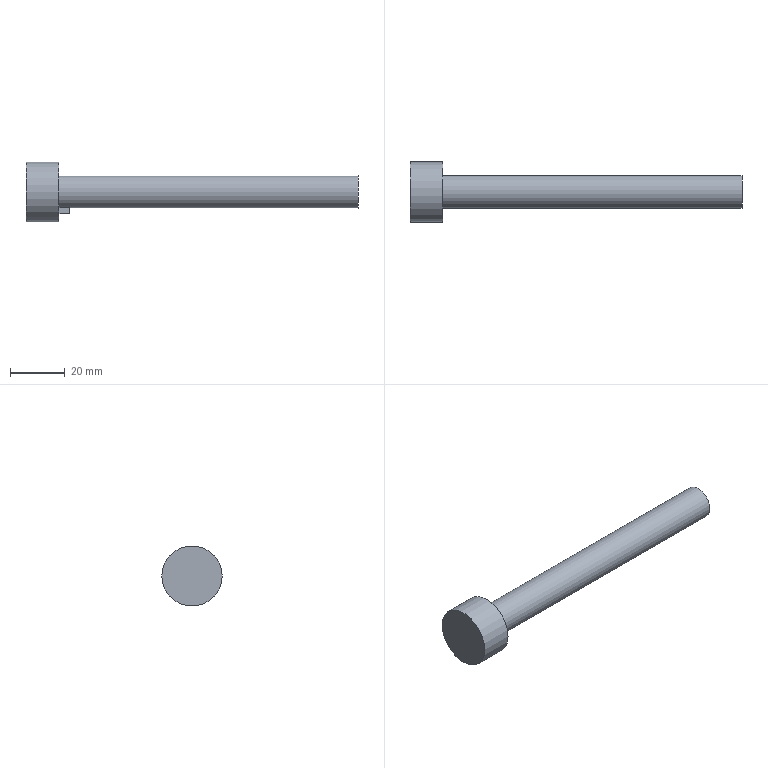Component | NX | BOLT_M12 | 2 solids | 11 faces | box 121 x 22 x 22 mm | volume 16923 mm3 | plane 8 | cylinder 3 | commonest cylinder face diameters 12 x2 22 x1
STEP:
#1=CARTESIAN_POINT('',(0.,0.,0.));
#2=DIRECTION('',(0.,0.,1.));
#3=DIRECTION('',(1.,0.,0.));
#4=AXIS2_PLACEMENT_3D('',#1,#2,#3);
#5=CARTESIAN_POINT('',(16.,11.,-95.));
#6=VERTEX_POINT('',#5);
#7=CARTESIAN_POINT('',(16.,0.,-95.));
#8=DIRECTION('',(-1.,0.,0.));
#9=DIRECTION('',(0.,1.,0.));
#10=AXIS2_PLACEMENT_3D('',#7,#8,#9);
#11=CIRCLE('',#10,11.);
#12=CARTESIAN_POINT('',(16.,0.,-95.));
#13=DIRECTION('',(-1.,0.,0.));
#14=DIRECTION('',(0.,0.,1.));
#15=AXIS2_PLACEMENT_3D('',#12,#13,#14);
#16=PLANE('',#15);
#17=CARTESIAN_POINT('',(0.,0.));
#18=DIRECTION('',(0.,1.));
#19=AXIS2_PLACEMENT_2D('',#17,#18);
#20=CIRCLE('',#19,11.);
#21=(GEOMETRIC_REPRESENTATION_CONTEXT(2)PARAMETRIC_REPRESENTATION_CONTEXT()REPRESENTATION_CONTEXT('',''));
#22=DEFINITIONAL_REPRESENTATION('',(#20),#21);
#23=PCURVE('',#16,#22);
#24=CARTESIAN_POINT('',(4.,0.,-95.));
#25=DIRECTION('',(1.,0.,0.));
#26=DIRECTION('',(0.,0.,-1.));
#27=AXIS2_PLACEMENT_3D('',#24,#25,#26);
#28=CYLINDRICAL_SURFACE('',#27,11.);
#29=CARTESIAN_POINT('',(7.854,12.));
#30=DIRECTION('',(-1.,0.));
#31=VECTOR('',#30,1.);
#32=LINE('',#29,#31);
#33=(GEOMETRIC_REPRESENTATION_CONTEXT(2)PARAMETRIC_REPRESENTATION_CONTEXT()REPRESENTATION_CONTEXT('',''));
#34=DEFINITIONAL_REPRESENTATION('',(#32),#33);
#35=PCURVE('',#28,#34);
#36=SURFACE_CURVE('',#11,(#23,#35),.PCURVE_S1.);
#37=EDGE_CURVE('',#6,#6,#36,.T.);
#38=ORIENTED_EDGE('',*,*,#37,.F.);
#39=EDGE_LOOP('',(#38));
#40=FACE_BOUND('',#39,.T.);
#41=CARTESIAN_POINT('',(16.,6.,-95.));
#42=VERTEX_POINT('',#41);
#43=CARTESIAN_POINT('',(16.,0.,-95.));
#44=DIRECTION('',(1.,0.,0.));
#45=DIRECTION('',(0.,1.,0.));
#46=AXIS2_PLACEMENT_3D('',#43,#44,#45);
#47=CIRCLE('',#46,6.);
#48=CARTESIAN_POINT('',(0.,6.));
#49=CARTESIAN_POINT('',(10.392,6.));
#50=CARTESIAN_POINT('',(5.196,-3.));
#51=CARTESIAN_POINT('',(0.,-12.));
#52=CARTESIAN_POINT('',(-5.196,-3.));
#53=CARTESIAN_POINT('',(-10.392,6.));
#54=CARTESIAN_POINT('',(0.,6.));
#55=(BOUNDED_CURVE()B_SPLINE_CURVE(2,(#48,#49,#50,#51,#52,#53,#54),.UNSPECIFIED.,.T.,.F.)B_SPLINE_CURVE_WITH_KNOTS((1,2,2,2,2,1),(-2.094,0.,2.094,4.189,6.283,8.378),.UNSPECIFIED.)CURVE()GEOMETRIC_REPRESENTATION_ITEM()RATIONAL_B_SPLINE_CURVE((1.,0.5,1.,0.5,1.,0.5,1.))REPRESENTATION_ITEM(''));
#56=(GEOMETRIC_REPRESENTATION_CONTEXT(2)PARAMETRIC_REPRESENTATION_CONTEXT()REPRESENTATION_CONTEXT('',''));
#57=DEFINITIONAL_REPRESENTATION('',(#55),#56);
#58=PCURVE('',#16,#57);
#59=CARTESIAN_POINT('',(125.,0.,-95.));
#60=DIRECTION('',(-1.,0.,0.));
#61=DIRECTION('',(0.,0.,1.));
#62=AXIS2_PLACEMENT_3D('',#59,#60,#61);
#63=CYLINDRICAL_SURFACE('',#62,6.);
#64=CARTESIAN_POINT('',(7.854,109.));
#65=DIRECTION('',(-1.,0.));
#66=VECTOR('',#65,1.);
#67=LINE('',#64,#66);
#68=(GEOMETRIC_REPRESENTATION_CONTEXT(2)PARAMETRIC_REPRESENTATION_CONTEXT()REPRESENTATION_CONTEXT('',''));
#69=DEFINITIONAL_REPRESENTATION('',(#67),#68);
#70=PCURVE('',#63,#69);
#71=SURFACE_CURVE('',#47,(#58,#70),.PCURVE_S1.);
#72=EDGE_CURVE('',#42,#42,#71,.T.);
#73=ORIENTED_EDGE('',*,*,#72,.F.);
#74=EDGE_LOOP('',(#73));
#75=FACE_BOUND('',#74,.T.);
#76=ADVANCED_FACE('',(#40,#75),#16,.F.);
#77=CARTESIAN_POINT('',(4.,11.,-95.));
#78=VERTEX_POINT('',#77);
#79=CARTESIAN_POINT('',(4.,0.,-95.));
#80=DIRECTION('',(-1.,0.,0.));
#81=DIRECTION('',(0.,1.,0.));
#82=AXIS2_PLACEMENT_3D('',#79,#80,#81);
#83=CIRCLE('',#82,11.);
#84=CARTESIAN_POINT('',(7.854,0.));
#85=DIRECTION('',(-1.,0.));
#86=VECTOR('',#85,1.);
#87=LINE('',#84,#86);
#88=(GEOMETRIC_REPRESENTATION_CONTEXT(2)PARAMETRIC_REPRESENTATION_CONTEXT()REPRESENTATION_CONTEXT('',''));
#89=DEFINITIONAL_REPRESENTATION('',(#87),#88);
#90=PCURVE('',#28,#89);
#91=CARTESIAN_POINT('',(4.,0.,-95.));
#92=DIRECTION('',(-1.,0.,0.));
#93=DIRECTION('',(0.,0.,1.));
#94=AXIS2_PLACEMENT_3D('',#91,#92,#93);
#95=PLANE('',#94);
#96=CARTESIAN_POINT('',(0.,0.));
#97=DIRECTION('',(0.,1.));
#98=AXIS2_PLACEMENT_2D('',#96,#97);
#99=CIRCLE('',#98,11.);
#100=(GEOMETRIC_REPRESENTATION_CONTEXT(2)PARAMETRIC_REPRESENTATION_CONTEXT()REPRESENTATION_CONTEXT('',''));
#101=DEFINITIONAL_REPRESENTATION('',(#99),#100);
#102=PCURVE('',#95,#101);
#103=SURFACE_CURVE('',#83,(#90,#102),.PCURVE_S1.);
#104=EDGE_CURVE('',#78,#78,#103,.T.);
#105=ORIENTED_EDGE('',*,*,#104,.F.);
#106=CARTESIAN_POINT('',(4.,11.,-95.));
#107=CARTESIAN_POINT('',(16.,11.,-95.));
#108=B_SPLINE_CURVE_WITH_KNOTS('',1,(#106,#107),.UNSPECIFIED.,.F.,.F.,(2,2),(0.,12.),.PIECEWISE_BEZIER_KNOTS.);
#109=CARTESIAN_POINT('',(7.854,0.));
#110=DIRECTION('',(0.,1.));
#111=VECTOR('',#110,1.);
#112=LINE('',#109,#111);
#113=(GEOMETRIC_REPRESENTATION_CONTEXT(2)PARAMETRIC_REPRESENTATION_CONTEXT()REPRESENTATION_CONTEXT('',''));
#114=DEFINITIONAL_REPRESENTATION('',(#112),#113);
#115=PCURVE('',#28,#114);
#116=CARTESIAN_POINT('',(1.571,0.));
#117=DIRECTION('',(0.,1.));
#118=VECTOR('',#117,1.);
#119=LINE('',#116,#118);
#120=(GEOMETRIC_REPRESENTATION_CONTEXT(2)PARAMETRIC_REPRESENTATION_CONTEXT()REPRESENTATION_CONTEXT('',''));
#121=DEFINITIONAL_REPRESENTATION('',(#119),#120);
#122=PCURVE('',#28,#121);
#123=SEAM_CURVE('',#108,(#115,#122),.PCURVE_S1.);
#124=EDGE_CURVE('',#78,#6,#123,.T.);
#125=ORIENTED_EDGE('',*,*,#124,.T.);
#126=ORIENTED_EDGE('',*,*,#37,.T.);
#127=ORIENTED_EDGE('',*,*,#124,.F.);
#128=EDGE_LOOP('',(#105,#125,#126,#127));
#129=FACE_BOUND('',#128,.T.);
#130=ADVANCED_FACE('',(#129),#28,.T.);
#131=ORIENTED_EDGE('',*,*,#104,.T.);
#132=EDGE_LOOP('',(#131));
#133=FACE_BOUND('',#132,.T.);
#134=ADVANCED_FACE('',(#133),#95,.T.);
#135=CARTESIAN_POINT('',(125.,6.,-95.));
#136=VERTEX_POINT('',#135);
#137=CARTESIAN_POINT('',(125.,0.,-95.));
#138=DIRECTION('',(1.,0.,0.));
#139=DIRECTION('',(0.,1.,0.));
#140=AXIS2_PLACEMENT_3D('',#137,#138,#139);
#141=CIRCLE('',#140,6.);
#142=CARTESIAN_POINT('',(7.854,0.));
#143=DIRECTION('',(-1.,0.));
#144=VECTOR('',#143,1.);
#145=LINE('',#142,#144);
#146=(GEOMETRIC_REPRESENTATION_CONTEXT(2)PARAMETRIC_REPRESENTATION_CONTEXT()REPRESENTATION_CONTEXT('',''));
#147=DEFINITIONAL_REPRESENTATION('',(#145),#146);
#148=PCURVE('',#63,#147);
#149=CARTESIAN_POINT('',(125.,0.,-95.));
#150=DIRECTION('',(1.,0.,0.));
#151=DIRECTION('',(0.,0.,-1.));
#152=AXIS2_PLACEMENT_3D('',#149,#150,#151);
#153=PLANE('',#152);
#154=CARTESIAN_POINT('',(0.,0.));
#155=DIRECTION('',(0.,1.));
#156=AXIS2_PLACEMENT_2D('',#154,#155);
#157=CIRCLE('',#156,6.);
#158=(GEOMETRIC_REPRESENTATION_CONTEXT(2)PARAMETRIC_REPRESENTATION_CONTEXT()REPRESENTATION_CONTEXT('',''));
#159=DEFINITIONAL_REPRESENTATION('',(#157),#158);
#160=PCURVE('',#153,#159);
#161=SURFACE_CURVE('',#141,(#148,#160),.PCURVE_S1.);
#162=EDGE_CURVE('',#136,#136,#161,.T.);
#163=ORIENTED_EDGE('',*,*,#162,.F.);
#164=CARTESIAN_POINT('',(125.,6.,-95.));
#165=CARTESIAN_POINT('',(16.,6.,-95.));
#166=B_SPLINE_CURVE_WITH_KNOTS('',1,(#164,#165),.UNSPECIFIED.,.F.,.F.,(2,2),(0.,109.),.PIECEWISE_BEZIER_KNOTS.);
#167=CARTESIAN_POINT('',(7.854,0.));
#168=DIRECTION('',(0.,1.));
#169=VECTOR('',#168,1.);
#170=LINE('',#167,#169);
#171=(GEOMETRIC_REPRESENTATION_CONTEXT(2)PARAMETRIC_REPRESENTATION_CONTEXT()REPRESENTATION_CONTEXT('',''));
#172=DEFINITIONAL_REPRESENTATION('',(#170),#171);
#173=PCURVE('',#63,#172);
#174=CARTESIAN_POINT('',(1.571,0.));
#175=DIRECTION('',(0.,1.));
#176=VECTOR('',#175,1.);
#177=LINE('',#174,#176);
#178=(GEOMETRIC_REPRESENTATION_CONTEXT(2)PARAMETRIC_REPRESENTATION_CONTEXT()REPRESENTATION_CONTEXT('',''));
#179=DEFINITIONAL_REPRESENTATION('',(#177),#178);
#180=PCURVE('',#63,#179);
#181=SEAM_CURVE('',#166,(#173,#180),.PCURVE_S1.);
#182=EDGE_CURVE('',#136,#42,#181,.T.);
#183=ORIENTED_EDGE('',*,*,#182,.T.);
#184=ORIENTED_EDGE('',*,*,#72,.T.);
#185=ORIENTED_EDGE('',*,*,#182,.F.);
#186=EDGE_LOOP('',(#163,#183,#184,#185));
#187=FACE_BOUND('',#186,.T.);
#188=ADVANCED_FACE('',(#187),#63,.T.);
#189=ORIENTED_EDGE('',*,*,#162,.T.);
#190=EDGE_LOOP('',(#189));
#191=FACE_BOUND('',#190,.T.);
#192=ADVANCED_FACE('',(#191),#153,.T.);
#193=CLOSED_SHELL('',(#76,#130,#134,#188,#192));
#194=MANIFOLD_SOLID_BREP('',#193);
#195=(LENGTH_UNIT()NAMED_UNIT(*)SI_UNIT(.MILLI.,.METRE.));
#196=UNCERTAINTY_MEASURE_WITH_UNIT(LENGTH_MEASURE(0.00001),#195,'','');
#197=(NAMED_UNIT(*)PLANE_ANGLE_UNIT()SI_UNIT($,.RADIAN.));
#198=(NAMED_UNIT(*)SI_UNIT($,.STERADIAN.)SOLID_ANGLE_UNIT());
#199=(GEOMETRIC_REPRESENTATION_CONTEXT(3)GLOBAL_UNCERTAINTY_ASSIGNED_CONTEXT((#196))GLOBAL_UNIT_ASSIGNED_CONTEXT((#195,#197,#198))REPRESENTATION_CONTEXT('',''));
#200=ADVANCED_BREP_SHAPE_REPRESENTATION('',(#4,#194),#199);
#201=CARTESIAN_POINT('',(0.,0.,0.));
#202=DIRECTION('',(0.,0.,1.));
#203=DIRECTION('',(1.,0.,0.));
#204=AXIS2_PLACEMENT_3D('',#201,#202,#203);
#205=CARTESIAN_POINT('',(0.,0.,0.));
#206=DIRECTION('',(0.,0.,1.));
#207=DIRECTION('',(1.,0.,0.));
#208=AXIS2_PLACEMENT_3D('',#205,#206,#207);
#209=(LENGTH_UNIT()NAMED_UNIT(*)SI_UNIT(.MILLI.,.METRE.));
#210=UNCERTAINTY_MEASURE_WITH_UNIT(LENGTH_MEASURE(0.000002),#209,'','');
#211=(NAMED_UNIT(*)PLANE_ANGLE_UNIT()SI_UNIT($,.RADIAN.));
#212=(NAMED_UNIT(*)SI_UNIT($,.STERADIAN.)SOLID_ANGLE_UNIT());
#213=(GEOMETRIC_REPRESENTATION_CONTEXT(3)GLOBAL_UNCERTAINTY_ASSIGNED_CONTEXT((#210))GLOBAL_UNIT_ASSIGNED_CONTEXT((#209,#211,#212))REPRESENTATION_CONTEXT('',''));
#214=SHAPE_REPRESENTATION('',(#4,#204,#208),#213);
#215=ITEM_DEFINED_TRANSFORMATION('','',#4,#204);
#216=(REPRESENTATION_RELATIONSHIP('','',#200,#214)REPRESENTATION_RELATIONSHIP_WITH_TRANSFORMATION(#215)SHAPE_REPRESENTATION_RELATIONSHIP());
#217=CARTESIAN_POINT('',(16.,-2.,-103.));
#218=VERTEX_POINT('',#217);
#219=CARTESIAN_POINT('',(16.,-2.,-100.657));
#220=VERTEX_POINT('',#219);
#221=CARTESIAN_POINT('',(16.,-2.,-103.));
#222=DIRECTION('',(0.,0.,1.));
#223=VECTOR('',#222,1.);
#224=LINE('',#221,#223);
#225=CARTESIAN_POINT('',(20.,-2.,-103.));
#226=DIRECTION('',(0.,-1.,0.));
#227=DIRECTION('',(0.,0.,1.));
#228=AXIS2_PLACEMENT_3D('',#225,#226,#227);
#229=PLANE('',#228);
#230=CARTESIAN_POINT('',(0.,4.));
#231=DIRECTION('',(1.,0.));
#232=VECTOR('',#231,1.);
#233=LINE('',#230,#232);
#234=(GEOMETRIC_REPRESENTATION_CONTEXT(2)PARAMETRIC_REPRESENTATION_CONTEXT()REPRESENTATION_CONTEXT('',''));
#235=DEFINITIONAL_REPRESENTATION('',(#233),#234);
#236=PCURVE('',#229,#235);
#237=CARTESIAN_POINT('',(16.,0.,-95.));
#238=DIRECTION('',(1.,0.,0.));
#239=DIRECTION('',(0.,0.,-1.));
#240=AXIS2_PLACEMENT_3D('',#237,#238,#239);
#241=PLANE('',#240);
#242=CARTESIAN_POINT('',(8.,-2.));
#243=DIRECTION('',(-1.,0.));
#244=VECTOR('',#243,1.);
#245=LINE('',#242,#244);
#246=(GEOMETRIC_REPRESENTATION_CONTEXT(2)PARAMETRIC_REPRESENTATION_CONTEXT()REPRESENTATION_CONTEXT('',''));
#247=DEFINITIONAL_REPRESENTATION('',(#245),#246);
#248=PCURVE('',#241,#247);
#249=SURFACE_CURVE('',#224,(#236,#248),.PCURVE_S1.);
#250=EDGE_CURVE('',#218,#220,#249,.T.);
#251=ORIENTED_EDGE('',*,*,#250,.F.);
#252=CARTESIAN_POINT('',(20.,-2.,-103.));
#253=VERTEX_POINT('',#252);
#254=CARTESIAN_POINT('',(20.,-2.,-103.));
#255=DIRECTION('',(-1.,0.,0.));
#256=VECTOR('',#255,1.);
#257=LINE('',#254,#256);
#258=CARTESIAN_POINT('',(0.,0.));
#259=DIRECTION('',(0.,1.));
#260=VECTOR('',#259,1.);
#261=LINE('',#258,#260);
#262=(GEOMETRIC_REPRESENTATION_CONTEXT(2)PARAMETRIC_REPRESENTATION_CONTEXT()REPRESENTATION_CONTEXT('',''));
#263=DEFINITIONAL_REPRESENTATION('',(#261),#262);
#264=PCURVE('',#229,#263);
#265=CARTESIAN_POINT('',(20.,2.,-103.));
#266=DIRECTION('',(0.,0.,-1.));
#267=DIRECTION('',(-1.,0.,0.));
#268=AXIS2_PLACEMENT_3D('',#265,#266,#267);
#269=PLANE('',#268);
#270=CARTESIAN_POINT('',(0.,-4.));
#271=DIRECTION('',(1.,0.));
#272=VECTOR('',#271,1.);
#273=LINE('',#270,#272);
#274=(GEOMETRIC_REPRESENTATION_CONTEXT(2)PARAMETRIC_REPRESENTATION_CONTEXT()REPRESENTATION_CONTEXT('',''));
#275=DEFINITIONAL_REPRESENTATION('',(#273),#274);
#276=PCURVE('',#269,#275);
#277=SURFACE_CURVE('',#257,(#264,#276),.PCURVE_S1.);
#278=EDGE_CURVE('',#253,#218,#277,.T.);
#279=ORIENTED_EDGE('',*,*,#278,.F.);
#280=CARTESIAN_POINT('',(20.,-2.,-100.657));
#281=VERTEX_POINT('',#280);
#282=CARTESIAN_POINT('',(20.,-2.,-103.));
#283=DIRECTION('',(0.,0.,1.));
#284=VECTOR('',#283,1.);
#285=LINE('',#282,#284);
#286=CARTESIAN_POINT('',(0.,0.));
#287=DIRECTION('',(1.,0.));
#288=VECTOR('',#287,1.);
#289=LINE('',#286,#288);
#290=(GEOMETRIC_REPRESENTATION_CONTEXT(2)PARAMETRIC_REPRESENTATION_CONTEXT()REPRESENTATION_CONTEXT('',''));
#291=DEFINITIONAL_REPRESENTATION('',(#289),#290);
#292=PCURVE('',#229,#291);
#293=CARTESIAN_POINT('',(20.,0.,-95.));
#294=DIRECTION('',(1.,0.,0.));
#295=DIRECTION('',(0.,0.,-1.));
#296=AXIS2_PLACEMENT_3D('',#293,#294,#295);
#297=PLANE('',#296);
#298=CARTESIAN_POINT('',(8.,-2.));
#299=DIRECTION('',(-1.,0.));
#300=VECTOR('',#299,1.);
#301=LINE('',#298,#300);
#302=(GEOMETRIC_REPRESENTATION_CONTEXT(2)PARAMETRIC_REPRESENTATION_CONTEXT()REPRESENTATION_CONTEXT('',''));
#303=DEFINITIONAL_REPRESENTATION('',(#301),#302);
#304=PCURVE('',#297,#303);
#305=SURFACE_CURVE('',#285,(#292,#304),.PCURVE_S1.);
#306=EDGE_CURVE('',#253,#281,#305,.T.);
#307=ORIENTED_EDGE('',*,*,#306,.T.);
#308=CARTESIAN_POINT('',(20.,-2.,-100.657));
#309=DIRECTION('',(-1.,0.,0.));
#310=VECTOR('',#309,1.);
#311=LINE('',#308,#310);
#312=CARTESIAN_POINT('',(2.343,0.));
#313=DIRECTION('',(0.,1.));
#314=VECTOR('',#313,1.);
#315=LINE('',#312,#314);
#316=(GEOMETRIC_REPRESENTATION_CONTEXT(2)PARAMETRIC_REPRESENTATION_CONTEXT()REPRESENTATION_CONTEXT('',''));
#317=DEFINITIONAL_REPRESENTATION('',(#315),#316);
#318=PCURVE('',#229,#317);
#319=CARTESIAN_POINT('',(20.,0.,-95.));
#320=DIRECTION('',(-1.,0.,0.));
#321=DIRECTION('',(0.,0.,1.));
#322=AXIS2_PLACEMENT_3D('',#319,#320,#321);
#323=CYLINDRICAL_SURFACE('',#322,6.);
#324=CARTESIAN_POINT('',(3.481,0.));
#325=DIRECTION('',(0.,1.));
#326=VECTOR('',#325,1.);
#327=LINE('',#324,#326);
#328=(GEOMETRIC_REPRESENTATION_CONTEXT(2)PARAMETRIC_REPRESENTATION_CONTEXT()REPRESENTATION_CONTEXT('',''));
#329=DEFINITIONAL_REPRESENTATION('',(#327),#328);
#330=PCURVE('',#323,#329);
#331=SURFACE_CURVE('',#311,(#318,#330),.PCURVE_S1.);
#332=EDGE_CURVE('',#281,#220,#331,.T.);
#333=ORIENTED_EDGE('',*,*,#332,.T.);
#334=EDGE_LOOP('',(#251,#279,#307,#333));
#335=FACE_BOUND('',#334,.T.);
#336=ADVANCED_FACE('',(#335),#229,.T.);
#337=CARTESIAN_POINT('',(20.,2.,-100.657));
#338=VERTEX_POINT('',#337);
#339=CARTESIAN_POINT('',(16.,2.,-100.657));
#340=VERTEX_POINT('',#339);
#341=CARTESIAN_POINT('',(20.,2.,-100.657));
#342=DIRECTION('',(-1.,0.,0.));
#343=VECTOR('',#342,1.);
#344=LINE('',#341,#343);
#345=CARTESIAN_POINT('',(2.802,0.));
#346=DIRECTION('',(0.,1.));
#347=VECTOR('',#346,1.);
#348=LINE('',#345,#347);
#349=(GEOMETRIC_REPRESENTATION_CONTEXT(2)PARAMETRIC_REPRESENTATION_CONTEXT()REPRESENTATION_CONTEXT('',''));
#350=DEFINITIONAL_REPRESENTATION('',(#348),#349);
#351=PCURVE('',#323,#350);
#352=CARTESIAN_POINT('',(20.,2.,-100.657));
#353=DIRECTION('',(0.,1.,0.));
#354=DIRECTION('',(0.,0.,-1.));
#355=AXIS2_PLACEMENT_3D('',#352,#353,#354);
#356=PLANE('',#355);
#357=CARTESIAN_POINT('',(-0.,0.));
#358=DIRECTION('',(0.,1.));
#359=VECTOR('',#358,1.);
#360=LINE('',#357,#359);
#361=(GEOMETRIC_REPRESENTATION_CONTEXT(2)PARAMETRIC_REPRESENTATION_CONTEXT()REPRESENTATION_CONTEXT('',''));
#362=DEFINITIONAL_REPRESENTATION('',(#360),#361);
#363=PCURVE('',#356,#362);
#364=SURFACE_CURVE('',#344,(#351,#363),.PCURVE_S1.);
#365=EDGE_CURVE('',#338,#340,#364,.T.);
#366=ORIENTED_EDGE('',*,*,#365,.F.);
#367=CARTESIAN_POINT('',(20.,0.,-95.));
#368=DIRECTION('',(1.,0.,0.));
#369=DIRECTION('',(0.,1.,0.));
#370=AXIS2_PLACEMENT_3D('',#367,#368,#369);
#371=CIRCLE('',#370,6.);
#372=CARTESIAN_POINT('',(7.854,0.));
#373=DIRECTION('',(-1.,0.));
#374=VECTOR('',#373,1.);
#375=LINE('',#372,#374);
#376=(GEOMETRIC_REPRESENTATION_CONTEXT(2)PARAMETRIC_REPRESENTATION_CONTEXT()REPRESENTATION_CONTEXT('',''));
#377=DEFINITIONAL_REPRESENTATION('',(#375),#376);
#378=PCURVE('',#323,#377);
#379=CARTESIAN_POINT('',(0.,0.));
#380=DIRECTION('',(0.,1.));
#381=AXIS2_PLACEMENT_2D('',#379,#380);
#382=CIRCLE('',#381,6.);
#383=(GEOMETRIC_REPRESENTATION_CONTEXT(2)PARAMETRIC_REPRESENTATION_CONTEXT()REPRESENTATION_CONTEXT('',''));
#384=DEFINITIONAL_REPRESENTATION('',(#382),#383);
#385=PCURVE('',#297,#384);
#386=SURFACE_CURVE('',#371,(#378,#385),.PCURVE_S1.);
#387=EDGE_CURVE('',#281,#338,#386,.T.);
#388=ORIENTED_EDGE('',*,*,#387,.F.);
#389=ORIENTED_EDGE('',*,*,#332,.T.);
#390=CARTESIAN_POINT('',(16.,0.,-95.));
#391=DIRECTION('',(1.,0.,0.));
#392=DIRECTION('',(0.,1.,0.));
#393=AXIS2_PLACEMENT_3D('',#390,#391,#392);
#394=CIRCLE('',#393,6.);
#395=CARTESIAN_POINT('',(7.854,4.));
#396=DIRECTION('',(-1.,0.));
#397=VECTOR('',#396,1.);
#398=LINE('',#395,#397);
#399=(GEOMETRIC_REPRESENTATION_CONTEXT(2)PARAMETRIC_REPRESENTATION_CONTEXT()REPRESENTATION_CONTEXT('',''));
#400=DEFINITIONAL_REPRESENTATION('',(#398),#399);
#401=PCURVE('',#323,#400);
#402=CARTESIAN_POINT('',(0.,0.));
#403=DIRECTION('',(0.,1.));
#404=AXIS2_PLACEMENT_2D('',#402,#403);
#405=CIRCLE('',#404,6.);
#406=(GEOMETRIC_REPRESENTATION_CONTEXT(2)PARAMETRIC_REPRESENTATION_CONTEXT()REPRESENTATION_CONTEXT('',''));
#407=DEFINITIONAL_REPRESENTATION('',(#405),#406);
#408=PCURVE('',#241,#407);
#409=SURFACE_CURVE('',#394,(#401,#408),.PCURVE_S1.);
#410=EDGE_CURVE('',#220,#340,#409,.T.);
#411=ORIENTED_EDGE('',*,*,#410,.T.);
#412=EDGE_LOOP('',(#366,#388,#389,#411));
#413=FACE_BOUND('',#412,.F.);
#414=ADVANCED_FACE('',(#413),#323,.F.);
#415=CARTESIAN_POINT('',(16.,2.,-103.));
#416=VERTEX_POINT('',#415);
#417=CARTESIAN_POINT('',(16.,2.,-100.657));
#418=DIRECTION('',(0.,0.,-1.));
#419=VECTOR('',#418,1.);
#420=LINE('',#417,#419);
#421=CARTESIAN_POINT('',(0.,4.));
#422=DIRECTION('',(1.,0.));
#423=VECTOR('',#422,1.);
#424=LINE('',#421,#423);
#425=(GEOMETRIC_REPRESENTATION_CONTEXT(2)PARAMETRIC_REPRESENTATION_CONTEXT()REPRESENTATION_CONTEXT('',''));
#426=DEFINITIONAL_REPRESENTATION('',(#424),#425);
#427=PCURVE('',#356,#426);
#428=CARTESIAN_POINT('',(5.657,2.));
#429=DIRECTION('',(1.,0.));
#430=VECTOR('',#429,1.);
#431=LINE('',#428,#430);
#432=(GEOMETRIC_REPRESENTATION_CONTEXT(2)PARAMETRIC_REPRESENTATION_CONTEXT()REPRESENTATION_CONTEXT('',''));
#433=DEFINITIONAL_REPRESENTATION('',(#431),#432);
#434=PCURVE('',#241,#433);
#435=SURFACE_CURVE('',#420,(#427,#434),.PCURVE_S1.);
#436=EDGE_CURVE('',#340,#416,#435,.T.);
#437=ORIENTED_EDGE('',*,*,#436,.F.);
#438=ORIENTED_EDGE('',*,*,#365,.F.);
#439=CARTESIAN_POINT('',(20.,2.,-103.));
#440=VERTEX_POINT('',#439);
#441=CARTESIAN_POINT('',(20.,2.,-100.657));
#442=DIRECTION('',(0.,0.,-1.));
#443=VECTOR('',#442,1.);
#444=LINE('',#441,#443);
#445=CARTESIAN_POINT('',(0.,0.));
#446=DIRECTION('',(1.,0.));
#447=VECTOR('',#446,1.);
#448=LINE('',#445,#447);
#449=(GEOMETRIC_REPRESENTATION_CONTEXT(2)PARAMETRIC_REPRESENTATION_CONTEXT()REPRESENTATION_CONTEXT('',''));
#450=DEFINITIONAL_REPRESENTATION('',(#448),#449);
#451=PCURVE('',#356,#450);
#452=CARTESIAN_POINT('',(5.657,2.));
#453=DIRECTION('',(1.,0.));
#454=VECTOR('',#453,1.);
#455=LINE('',#452,#454);
#456=(GEOMETRIC_REPRESENTATION_CONTEXT(2)PARAMETRIC_REPRESENTATION_CONTEXT()REPRESENTATION_CONTEXT('',''));
#457=DEFINITIONAL_REPRESENTATION('',(#455),#456);
#458=PCURVE('',#297,#457);
#459=SURFACE_CURVE('',#444,(#451,#458),.PCURVE_S1.);
#460=EDGE_CURVE('',#338,#440,#459,.T.);
#461=ORIENTED_EDGE('',*,*,#460,.T.);
#462=CARTESIAN_POINT('',(20.,2.,-103.));
#463=DIRECTION('',(-1.,0.,0.));
#464=VECTOR('',#463,1.);
#465=LINE('',#462,#464);
#466=CARTESIAN_POINT('',(2.343,0.));
#467=DIRECTION('',(0.,1.));
#468=VECTOR('',#467,1.);
#469=LINE('',#466,#468);
#470=(GEOMETRIC_REPRESENTATION_CONTEXT(2)PARAMETRIC_REPRESENTATION_CONTEXT()REPRESENTATION_CONTEXT('',''));
#471=DEFINITIONAL_REPRESENTATION('',(#469),#470);
#472=PCURVE('',#356,#471);
#473=CARTESIAN_POINT('',(0.,0.));
#474=DIRECTION('',(1.,0.));
#475=VECTOR('',#474,1.);
#476=LINE('',#473,#475);
#477=(GEOMETRIC_REPRESENTATION_CONTEXT(2)PARAMETRIC_REPRESENTATION_CONTEXT()REPRESENTATION_CONTEXT('',''));
#478=DEFINITIONAL_REPRESENTATION('',(#476),#477);
#479=PCURVE('',#269,#478);
#480=SURFACE_CURVE('',#465,(#472,#479),.PCURVE_S1.);
#481=EDGE_CURVE('',#440,#416,#480,.T.);
#482=ORIENTED_EDGE('',*,*,#481,.T.);
#483=EDGE_LOOP('',(#437,#438,#461,#482));
#484=FACE_BOUND('',#483,.T.);
#485=ADVANCED_FACE('',(#484),#356,.T.);
#486=CARTESIAN_POINT('',(16.,2.,-103.));
#487=DIRECTION('',(0.,-1.,0.));
#488=VECTOR('',#487,1.);
#489=LINE('',#486,#488);
#490=CARTESIAN_POINT('',(4.,0.));
#491=DIRECTION('',(0.,-1.));
#492=VECTOR('',#491,1.);
#493=LINE('',#490,#492);
#494=(GEOMETRIC_REPRESENTATION_CONTEXT(2)PARAMETRIC_REPRESENTATION_CONTEXT()REPRESENTATION_CONTEXT('',''));
#495=DEFINITIONAL_REPRESENTATION('',(#493),#494);
#496=PCURVE('',#269,#495);
#497=CARTESIAN_POINT('',(8.,2.));
#498=DIRECTION('',(0.,-1.));
#499=VECTOR('',#498,1.);
#500=LINE('',#497,#499);
#501=(GEOMETRIC_REPRESENTATION_CONTEXT(2)PARAMETRIC_REPRESENTATION_CONTEXT()REPRESENTATION_CONTEXT('',''));
#502=DEFINITIONAL_REPRESENTATION('',(#500),#501);
#503=PCURVE('',#241,#502);
#504=SURFACE_CURVE('',#489,(#496,#503),.PCURVE_S1.);
#505=EDGE_CURVE('',#416,#218,#504,.T.);
#506=ORIENTED_EDGE('',*,*,#505,.F.);
#507=ORIENTED_EDGE('',*,*,#481,.F.);
#508=CARTESIAN_POINT('',(20.,2.,-103.));
#509=DIRECTION('',(0.,-1.,0.));
#510=VECTOR('',#509,1.);
#511=LINE('',#508,#510);
#512=CARTESIAN_POINT('',(0.,0.));
#513=DIRECTION('',(0.,-1.));
#514=VECTOR('',#513,1.);
#515=LINE('',#512,#514);
#516=(GEOMETRIC_REPRESENTATION_CONTEXT(2)PARAMETRIC_REPRESENTATION_CONTEXT()REPRESENTATION_CONTEXT('',''));
#517=DEFINITIONAL_REPRESENTATION('',(#515),#516);
#518=PCURVE('',#269,#517);
#519=CARTESIAN_POINT('',(8.,2.));
#520=DIRECTION('',(0.,-1.));
#521=VECTOR('',#520,1.);
#522=LINE('',#519,#521);
#523=(GEOMETRIC_REPRESENTATION_CONTEXT(2)PARAMETRIC_REPRESENTATION_CONTEXT()REPRESENTATION_CONTEXT('',''));
#524=DEFINITIONAL_REPRESENTATION('',(#522),#523);
#525=PCURVE('',#297,#524);
#526=SURFACE_CURVE('',#511,(#518,#525),.PCURVE_S1.);
#527=EDGE_CURVE('',#440,#253,#526,.T.);
#528=ORIENTED_EDGE('',*,*,#527,.T.);
#529=ORIENTED_EDGE('',*,*,#278,.T.);
#530=EDGE_LOOP('',(#506,#507,#528,#529));
#531=FACE_BOUND('',#530,.T.);
#532=ADVANCED_FACE('',(#531),#269,.T.);
#533=ORIENTED_EDGE('',*,*,#306,.F.);
#534=ORIENTED_EDGE('',*,*,#527,.F.);
#535=ORIENTED_EDGE('',*,*,#460,.F.);
#536=ORIENTED_EDGE('',*,*,#387,.F.);
#537=EDGE_LOOP('',(#533,#534,#535,#536));
#538=FACE_BOUND('',#537,.T.);
#539=ADVANCED_FACE('',(#538),#297,.T.);
#540=ORIENTED_EDGE('',*,*,#250,.T.);
#541=ORIENTED_EDGE('',*,*,#410,.T.);
#542=ORIENTED_EDGE('',*,*,#436,.T.);
#543=ORIENTED_EDGE('',*,*,#505,.T.);
#544=EDGE_LOOP('',(#540,#541,#542,#543));
#545=FACE_BOUND('',#544,.T.);
#546=ADVANCED_FACE('',(#545),#241,.F.);
#547=CLOSED_SHELL('',(#336,#414,#485,#532,#539,#546));
#548=MANIFOLD_SOLID_BREP('',#547);
#549=(LENGTH_UNIT()NAMED_UNIT(*)SI_UNIT(.MILLI.,.METRE.));
#550=UNCERTAINTY_MEASURE_WITH_UNIT(LENGTH_MEASURE(0.0000001),#549,'','');
#551=(NAMED_UNIT(*)PLANE_ANGLE_UNIT()SI_UNIT($,.RADIAN.));
#552=(NAMED_UNIT(*)SI_UNIT($,.STERADIAN.)SOLID_ANGLE_UNIT());
#553=(GEOMETRIC_REPRESENTATION_CONTEXT(3)GLOBAL_UNCERTAINTY_ASSIGNED_CONTEXT((#550))GLOBAL_UNIT_ASSIGNED_CONTEXT((#549,#551,#552))REPRESENTATION_CONTEXT('',''));
#554=ADVANCED_BREP_SHAPE_REPRESENTATION('',(#4,#548),#553);
#555=ITEM_DEFINED_TRANSFORMATION('','',#4,#208);
#556=(REPRESENTATION_RELATIONSHIP('','',#554,#214)REPRESENTATION_RELATIONSHIP_WITH_TRANSFORMATION(#555)SHAPE_REPRESENTATION_RELATIONSHIP());